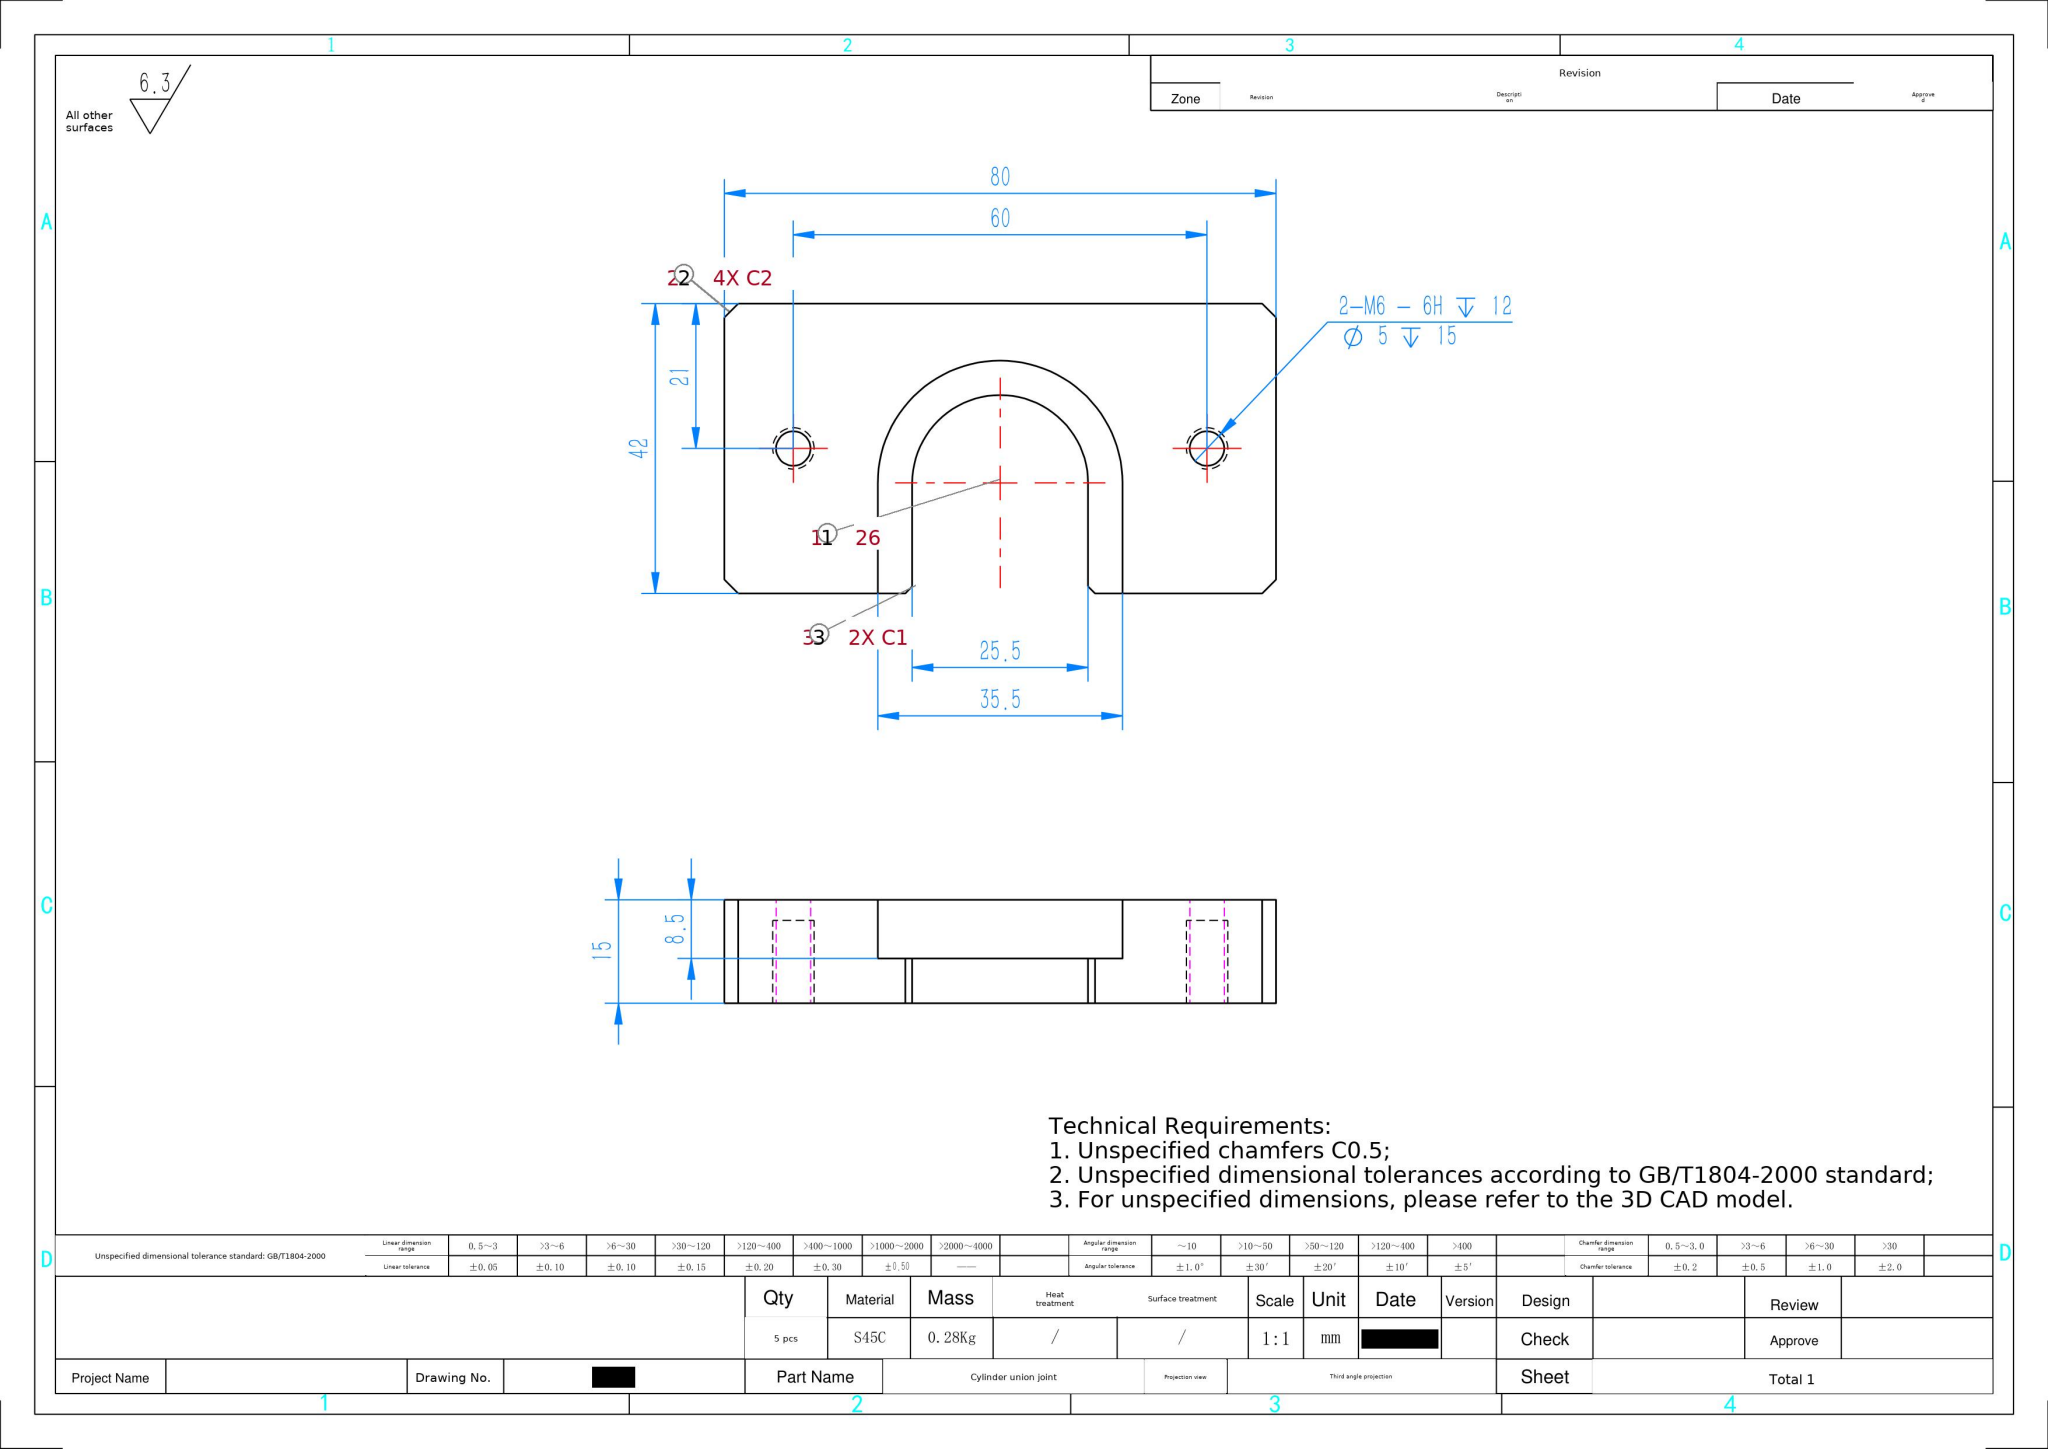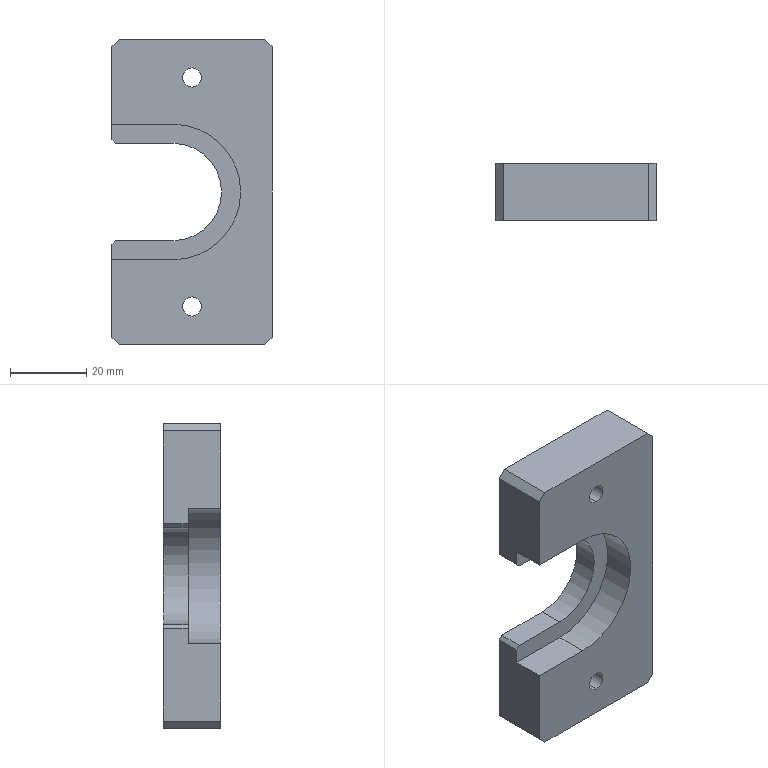Part | SolidWorks | mm | material S45C | 1 solid | 24 faces | box 42 x 15 x 80 mm | volume 36338 mm3 | plane 18 | cylinder 6 | commonest cylinder face diameters 5 x4 25.5 x1 35.5 x1
build123d program:
from build123d import *

# Parameters (mm, degrees)
SKETCH1_W             = 42
SKETCH1_H             = 80
BOSS_EXTRUDE1_DEPTH   = 15
CUT_EXTRUDE1_DEPTH    = 48.603
CUT_EXTRUDE2_DEPTH    = 8.5
M6_TAPPED_HOLE1_D     = 5
M6_TAPPED_HOLE1_DEPTH = 15
M6_TAPPED_HOLE1_TIP   = 1.502
CHAMFER1_SIZE         = 2
CHAMFER2_SIZE         = 1


with BuildPart() as part:
    # Sketch1 → Boss-Extrude1 (new body)
    with BuildSketch(Plane(origin=(0, 0, 0), x_dir=(1, 0, 0), z_dir=(0, 1, 0))):
        Rectangle(SKETCH1_W, SKETCH1_H)
    extrude(amount=BOSS_EXTRUDE1_DEPTH)

    # Sketch2 → Cut-Extrude1 (cut, through all)
    with BuildSketch(Plane(origin=(0, 15, 0), x_dir=(1, 0, 0), z_dir=(0, 1, 0))):
        with BuildLine():
            Line((-37, 12.75), (-5, 12.75))
            ThreePointArc((-5, 12.75), (7.75, 0), (-5, -12.75))
            Line((-5, -12.75), (-37, -12.75))
            ThreePointArc((-37, -12.75), (-49.75, 0), (-37, 12.75))
        make_face()
    extrude(amount=-CUT_EXTRUDE1_DEPTH, mode=Mode.SUBTRACT)

    # Sketch3 → Cut-Extrude2 (cut)
    with BuildSketch(Plane.XZ):
        with BuildLine():
            Line((-21, -17.75), (-21, 17.75))
            Line((-21, 17.75), (-5, 17.75))
            ThreePointArc((-5, 17.75), (12.75, 0), (-5, -17.75))
            Line((-5, -17.75), (-21, -17.75))
        make_face()
    extrude(amount=-CUT_EXTRUDE2_DEPTH, mode=Mode.SUBTRACT)

    # M6 Tapped Hole1
    with Locations(Plane(origin=(0, 15, 0), x_dir=(1, 0, 0), z_dir=(0, 1, 0))):
        with Locations((0, -30), (0, 30)):
            Hole(M6_TAPPED_HOLE1_D / 2, depth=M6_TAPPED_HOLE1_DEPTH)
            with Locations((0, 0, -(M6_TAPPED_HOLE1_DEPTH + M6_TAPPED_HOLE1_TIP / 2))):  # 118° drill point
                Cone(0, M6_TAPPED_HOLE1_D / 2, M6_TAPPED_HOLE1_TIP, mode=Mode.SUBTRACT)

    # Chamfer1
    chamfer1_edges = [part.edges().sort_by_distance(p)[0] for p in [
        (21, 7.5, 40),
        (-21, 7.5, 40),
        (-21, 7.5, -40),
        (21, 7.5, -40),
    ]]
    chamfer(chamfer1_edges, length=CHAMFER1_SIZE)

    # Chamfer2
    chamfer2_edges = [part.edges().sort_by_distance(p)[0] for p in [
        (-21, 11.75, 12.75),
        (-21, 11.75, -12.75),
    ]]
    chamfer(chamfer2_edges, length=CHAMFER2_SIZE)


solid = part.part
STEP:
#1=CARTESIAN_POINT('',(0.,0.,-32.5));
#2=VERTEX_POINT('',#1);
#3=CARTESIAN_POINT('',(0.,0.,-27.5));
#4=VERTEX_POINT('',#3);
#5=CARTESIAN_POINT('',(0.,0.,-30.));
#6=DIRECTION('',(0.,1.,0.));
#7=DIRECTION('',(0.,0.,1.));
#8=AXIS2_PLACEMENT_3D('',#5,#6,#7);
#9=CIRCLE('',#8,2.5);
#10=EDGE_CURVE('',#2,#4,#9,.T.);
#11=ORIENTED_EDGE('',*,*,#10,.F.);
#12=CARTESIAN_POINT('',(0.,15.,-32.5));
#13=VERTEX_POINT('',#12);
#14=CARTESIAN_POINT('',(0.,15.,-32.5));
#15=DIRECTION('',(0.,1.,0.));
#16=VECTOR('',#15,1000.);
#17=LINE('',#14,#16);
#18=EDGE_CURVE('',#2,#13,#17,.T.);
#19=ORIENTED_EDGE('',*,*,#18,.T.);
#20=CARTESIAN_POINT('',(0.,15.,-27.5));
#21=VERTEX_POINT('',#20);
#22=CARTESIAN_POINT('',(0.,15.,-30.));
#23=DIRECTION('',(0.,1.,0.));
#24=DIRECTION('',(0.,0.,1.));
#25=AXIS2_PLACEMENT_3D('',#22,#23,#24);
#26=CIRCLE('',#25,2.5);
#27=EDGE_CURVE('',#13,#21,#26,.T.);
#28=ORIENTED_EDGE('',*,*,#27,.T.);
#29=CARTESIAN_POINT('',(0.,15.,-27.5));
#30=DIRECTION('',(0.,1.,0.));
#31=VECTOR('',#30,1000.);
#32=LINE('',#29,#31);
#33=EDGE_CURVE('',#4,#21,#32,.T.);
#34=ORIENTED_EDGE('',*,*,#33,.F.);
#35=EDGE_LOOP('',(#11,#19,#28,#34));
#36=FACE_OUTER_BOUND('',#35,.T.);
#37=CARTESIAN_POINT('',(0.,15.,-30.));
#38=DIRECTION('',(0.,1.,0.));
#39=DIRECTION('',(0.,0.,1.));
#40=AXIS2_PLACEMENT_3D('',#37,#38,#39);
#41=CYLINDRICAL_SURFACE('',#40,2.5);
#42=ADVANCED_FACE('',(#36),#41,.F.);
#43=CARTESIAN_POINT('',(0.,0.,27.5));
#44=VERTEX_POINT('',#43);
#45=CARTESIAN_POINT('',(0.,0.,32.5));
#46=VERTEX_POINT('',#45);
#47=CARTESIAN_POINT('',(0.,0.,30.));
#48=DIRECTION('',(0.,1.,0.));
#49=DIRECTION('',(0.,0.,1.));
#50=AXIS2_PLACEMENT_3D('',#47,#48,#49);
#51=CIRCLE('',#50,2.5);
#52=EDGE_CURVE('',#44,#46,#51,.T.);
#53=ORIENTED_EDGE('',*,*,#52,.F.);
#54=CARTESIAN_POINT('',(0.,15.,27.5));
#55=VERTEX_POINT('',#54);
#56=CARTESIAN_POINT('',(0.,15.,27.5));
#57=DIRECTION('',(0.,1.,0.));
#58=VECTOR('',#57,1000.);
#59=LINE('',#56,#58);
#60=EDGE_CURVE('',#44,#55,#59,.T.);
#61=ORIENTED_EDGE('',*,*,#60,.T.);
#62=CARTESIAN_POINT('',(0.,15.,32.5));
#63=VERTEX_POINT('',#62);
#64=CARTESIAN_POINT('',(0.,15.,30.));
#65=DIRECTION('',(0.,1.,0.));
#66=DIRECTION('',(0.,0.,1.));
#67=AXIS2_PLACEMENT_3D('',#64,#65,#66);
#68=CIRCLE('',#67,2.5);
#69=EDGE_CURVE('',#55,#63,#68,.T.);
#70=ORIENTED_EDGE('',*,*,#69,.T.);
#71=CARTESIAN_POINT('',(0.,15.,32.5));
#72=DIRECTION('',(0.,1.,0.));
#73=VECTOR('',#72,1000.);
#74=LINE('',#71,#73);
#75=EDGE_CURVE('',#46,#63,#74,.T.);
#76=ORIENTED_EDGE('',*,*,#75,.F.);
#77=EDGE_LOOP('',(#53,#61,#70,#76));
#78=FACE_OUTER_BOUND('',#77,.T.);
#79=CARTESIAN_POINT('',(0.,15.,30.));
#80=DIRECTION('',(0.,1.,0.));
#81=DIRECTION('',(0.,0.,1.));
#82=AXIS2_PLACEMENT_3D('',#79,#80,#81);
#83=CYLINDRICAL_SURFACE('',#82,2.5);
#84=ADVANCED_FACE('',(#78),#83,.F.);
#85=CARTESIAN_POINT('',(-5.,15.,-12.75));
#86=VERTEX_POINT('',#85);
#87=CARTESIAN_POINT('',(-20.,15.,-12.75));
#88=VERTEX_POINT('',#87);
#89=CARTESIAN_POINT('',(-37.,15.,-12.75));
#90=DIRECTION('',(-1.,0.,0.));
#91=VECTOR('',#90,1000.);
#92=LINE('',#89,#91);
#93=EDGE_CURVE('',#86,#88,#92,.T.);
#94=ORIENTED_EDGE('',*,*,#93,.T.);
#95=CARTESIAN_POINT('',(-20.,8.5,-12.75));
#96=VERTEX_POINT('',#95);
#97=CARTESIAN_POINT('',(-20.,0.,-12.75));
#98=DIRECTION('',(0.,-1.,0.));
#99=VECTOR('',#98,1000.);
#100=LINE('',#97,#99);
#101=EDGE_CURVE('',#88,#96,#100,.T.);
#102=ORIENTED_EDGE('',*,*,#101,.T.);
#103=CARTESIAN_POINT('',(-5.,8.5,-12.75));
#104=VERTEX_POINT('',#103);
#105=CARTESIAN_POINT('',(-37.,8.5,-12.75));
#106=DIRECTION('',(-1.,0.,0.));
#107=VECTOR('',#106,1000.);
#108=LINE('',#105,#107);
#109=EDGE_CURVE('',#104,#96,#108,.T.);
#110=ORIENTED_EDGE('',*,*,#109,.F.);
#111=CARTESIAN_POINT('',(-5.,0.,-12.75));
#112=DIRECTION('',(0.,1.,0.));
#113=VECTOR('',#112,1000.);
#114=LINE('',#111,#113);
#115=EDGE_CURVE('',#104,#86,#114,.T.);
#116=ORIENTED_EDGE('',*,*,#115,.T.);
#117=EDGE_LOOP('',(#94,#102,#110,#116));
#118=FACE_OUTER_BOUND('',#117,.T.);
#119=CARTESIAN_POINT('',(-37.,0.,-12.75));
#120=DIRECTION('',(-0.,0.,-1.));
#121=DIRECTION('',(-1.,0.,0.));
#122=AXIS2_PLACEMENT_3D('',#119,#120,#121);
#123=PLANE('',#122);
#124=ADVANCED_FACE('',(#118),#123,.F.);
#125=CARTESIAN_POINT('',(-20.,8.5,12.75));
#126=VERTEX_POINT('',#125);
#127=CARTESIAN_POINT('',(-5.,8.5,12.75));
#128=VERTEX_POINT('',#127);
#129=CARTESIAN_POINT('',(-37.,8.5,12.75));
#130=DIRECTION('',(1.,0.,-0.));
#131=VECTOR('',#130,1000.);
#132=LINE('',#129,#131);
#133=EDGE_CURVE('',#126,#128,#132,.T.);
#134=ORIENTED_EDGE('',*,*,#133,.F.);
#135=CARTESIAN_POINT('',(-20.,15.,12.75));
#136=VERTEX_POINT('',#135);
#137=CARTESIAN_POINT('',(-20.,0.,12.75));
#138=DIRECTION('',(0.,1.,0.));
#139=VECTOR('',#138,1000.);
#140=LINE('',#137,#139);
#141=EDGE_CURVE('',#126,#136,#140,.T.);
#142=ORIENTED_EDGE('',*,*,#141,.T.);
#143=CARTESIAN_POINT('',(-5.,15.,12.75));
#144=VERTEX_POINT('',#143);
#145=CARTESIAN_POINT('',(-37.,15.,12.75));
#146=DIRECTION('',(1.,0.,-0.));
#147=VECTOR('',#146,1000.);
#148=LINE('',#145,#147);
#149=EDGE_CURVE('',#136,#144,#148,.T.);
#150=ORIENTED_EDGE('',*,*,#149,.T.);
#151=CARTESIAN_POINT('',(-5.,0.,12.75));
#152=DIRECTION('',(0.,1.,0.));
#153=VECTOR('',#152,1000.);
#154=LINE('',#151,#153);
#155=EDGE_CURVE('',#128,#144,#154,.T.);
#156=ORIENTED_EDGE('',*,*,#155,.F.);
#157=EDGE_LOOP('',(#134,#142,#150,#156));
#158=FACE_OUTER_BOUND('',#157,.T.);
#159=CARTESIAN_POINT('',(-37.,0.,12.75));
#160=DIRECTION('',(0.,0.,1.));
#161=DIRECTION('',(1.,0.,-0.));
#162=AXIS2_PLACEMENT_3D('',#159,#160,#161);
#163=PLANE('',#162);
#164=ADVANCED_FACE('',(#158),#163,.F.);
#165=CARTESIAN_POINT('',(-5.,8.5,-0.));
#166=DIRECTION('',(0.,1.,0.));
#167=DIRECTION('',(0.,0.,-1.));
#168=AXIS2_PLACEMENT_3D('',#165,#166,#167);
#169=CIRCLE('',#168,12.75);
#170=EDGE_CURVE('',#128,#104,#169,.T.);
#171=ORIENTED_EDGE('',*,*,#170,.F.);
#172=ORIENTED_EDGE('',*,*,#155,.T.);
#173=CARTESIAN_POINT('',(-5.,15.,-0.));
#174=DIRECTION('',(0.,1.,0.));
#175=DIRECTION('',(0.,0.,1.));
#176=AXIS2_PLACEMENT_3D('',#173,#174,#175);
#177=CIRCLE('',#176,12.75);
#178=EDGE_CURVE('',#144,#86,#177,.T.);
#179=ORIENTED_EDGE('',*,*,#178,.T.);
#180=ORIENTED_EDGE('',*,*,#115,.F.);
#181=EDGE_LOOP('',(#171,#172,#179,#180));
#182=FACE_OUTER_BOUND('',#181,.T.);
#183=CARTESIAN_POINT('',(-5.,0.,-0.));
#184=DIRECTION('',(0.,1.,0.));
#185=DIRECTION('',(0.,0.,1.));
#186=AXIS2_PLACEMENT_3D('',#183,#184,#185);
#187=CYLINDRICAL_SURFACE('',#186,12.75);
#188=ADVANCED_FACE('',(#182),#187,.F.);
#189=CARTESIAN_POINT('',(-21.,8.5,-13.75));
#190=VERTEX_POINT('',#189);
#191=CARTESIAN_POINT('',(-21.,8.5,-17.75));
#192=VERTEX_POINT('',#191);
#193=CARTESIAN_POINT('',(-21.,8.5,-17.75));
#194=DIRECTION('',(0.,0.,-1.));
#195=VECTOR('',#194,1000.);
#196=LINE('',#193,#195);
#197=EDGE_CURVE('',#190,#192,#196,.T.);
#198=ORIENTED_EDGE('',*,*,#197,.F.);
#199=CARTESIAN_POINT('',(-21.,15.,-13.75));
#200=VERTEX_POINT('',#199);
#201=CARTESIAN_POINT('',(-21.,15.,-13.75));
#202=DIRECTION('',(0.,1.,0.));
#203=VECTOR('',#202,1000.);
#204=LINE('',#201,#203);
#205=EDGE_CURVE('',#190,#200,#204,.T.);
#206=ORIENTED_EDGE('',*,*,#205,.T.);
#207=CARTESIAN_POINT('',(-21.,15.,-38.));
#208=VERTEX_POINT('',#207);
#209=CARTESIAN_POINT('',(-21.,15.,-40.));
#210=DIRECTION('',(0.,0.,1.));
#211=VECTOR('',#210,1000.);
#212=LINE('',#209,#211);
#213=EDGE_CURVE('',#208,#200,#212,.T.);
#214=ORIENTED_EDGE('',*,*,#213,.F.);
#215=CARTESIAN_POINT('',(-21.,0.,-38.));
#216=VERTEX_POINT('',#215);
#217=CARTESIAN_POINT('',(-21.,15.,-38.));
#218=DIRECTION('',(0.,-1.,0.));
#219=VECTOR('',#218,1000.);
#220=LINE('',#217,#219);
#221=EDGE_CURVE('',#208,#216,#220,.T.);
#222=ORIENTED_EDGE('',*,*,#221,.T.);
#223=CARTESIAN_POINT('',(-21.,0.,-17.75));
#224=VERTEX_POINT('',#223);
#225=CARTESIAN_POINT('',(-21.,0.,-40.));
#226=DIRECTION('',(0.,0.,1.));
#227=VECTOR('',#226,1000.);
#228=LINE('',#225,#227);
#229=EDGE_CURVE('',#216,#224,#228,.T.);
#230=ORIENTED_EDGE('',*,*,#229,.T.);
#231=CARTESIAN_POINT('',(-21.,8.5,-17.75));
#232=DIRECTION('',(0.,-1.,0.));
#233=VECTOR('',#232,1000.);
#234=LINE('',#231,#233);
#235=EDGE_CURVE('',#192,#224,#234,.T.);
#236=ORIENTED_EDGE('',*,*,#235,.F.);
#237=EDGE_LOOP('',(#198,#206,#214,#222,#230,#236));
#238=FACE_OUTER_BOUND('',#237,.T.);
#239=CARTESIAN_POINT('',(-21.,15.,-40.));
#240=DIRECTION('',(1.,0.,-0.));
#241=DIRECTION('',(-0.,0.,-1.));
#242=AXIS2_PLACEMENT_3D('',#239,#240,#241);
#243=PLANE('',#242);
#244=ADVANCED_FACE('',(#238),#243,.F.);
#245=CARTESIAN_POINT('',(21.,0.,38.));
#246=VERTEX_POINT('',#245);
#247=CARTESIAN_POINT('',(21.,0.,-38.));
#248=VERTEX_POINT('',#247);
#249=CARTESIAN_POINT('',(21.,0.,-40.));
#250=DIRECTION('',(-0.,0.,-1.));
#251=VECTOR('',#250,1000.);
#252=LINE('',#249,#251);
#253=EDGE_CURVE('',#246,#248,#252,.T.);
#254=ORIENTED_EDGE('',*,*,#253,.T.);
#255=CARTESIAN_POINT('',(21.,15.,-38.));
#256=VERTEX_POINT('',#255);
#257=CARTESIAN_POINT('',(21.,15.,-38.));
#258=DIRECTION('',(0.,1.,0.));
#259=VECTOR('',#258,1000.);
#260=LINE('',#257,#259);
#261=EDGE_CURVE('',#248,#256,#260,.T.);
#262=ORIENTED_EDGE('',*,*,#261,.T.);
#263=CARTESIAN_POINT('',(21.,15.,38.));
#264=VERTEX_POINT('',#263);
#265=CARTESIAN_POINT('',(21.,15.,-40.));
#266=DIRECTION('',(-0.,0.,-1.));
#267=VECTOR('',#266,1000.);
#268=LINE('',#265,#267);
#269=EDGE_CURVE('',#264,#256,#268,.T.);
#270=ORIENTED_EDGE('',*,*,#269,.F.);
#271=CARTESIAN_POINT('',(21.,15.,38.));
#272=DIRECTION('',(0.,-1.,0.));
#273=VECTOR('',#272,1000.);
#274=LINE('',#271,#273);
#275=EDGE_CURVE('',#264,#246,#274,.T.);
#276=ORIENTED_EDGE('',*,*,#275,.T.);
#277=EDGE_LOOP('',(#254,#262,#270,#276));
#278=FACE_OUTER_BOUND('',#277,.T.);
#279=CARTESIAN_POINT('',(21.,15.,-40.));
#280=DIRECTION('',(-1.,0.,0.));
#281=DIRECTION('',(0.,0.,1.));
#282=AXIS2_PLACEMENT_3D('',#279,#280,#281);
#283=PLANE('',#282);
#284=ADVANCED_FACE('',(#278),#283,.F.);
#285=CARTESIAN_POINT('',(19.,15.,-40.));
#286=VERTEX_POINT('',#285);
#287=CARTESIAN_POINT('',(-19.,15.,-40.));
#288=VERTEX_POINT('',#287);
#289=CARTESIAN_POINT('',(-21.,15.,-40.));
#290=DIRECTION('',(-1.,0.,0.));
#291=VECTOR('',#290,1000.);
#292=LINE('',#289,#291);
#293=EDGE_CURVE('',#286,#288,#292,.T.);
#294=ORIENTED_EDGE('',*,*,#293,.F.);
#295=CARTESIAN_POINT('',(19.,0.,-40.));
#296=VERTEX_POINT('',#295);
#297=CARTESIAN_POINT('',(19.,15.,-40.));
#298=DIRECTION('',(0.,-1.,0.));
#299=VECTOR('',#298,1000.);
#300=LINE('',#297,#299);
#301=EDGE_CURVE('',#286,#296,#300,.T.);
#302=ORIENTED_EDGE('',*,*,#301,.T.);
#303=CARTESIAN_POINT('',(-19.,0.,-40.));
#304=VERTEX_POINT('',#303);
#305=CARTESIAN_POINT('',(-21.,0.,-40.));
#306=DIRECTION('',(-1.,0.,0.));
#307=VECTOR('',#306,1000.);
#308=LINE('',#305,#307);
#309=EDGE_CURVE('',#296,#304,#308,.T.);
#310=ORIENTED_EDGE('',*,*,#309,.T.);
#311=CARTESIAN_POINT('',(-19.,15.,-40.));
#312=DIRECTION('',(0.,1.,0.));
#313=VECTOR('',#312,1000.);
#314=LINE('',#311,#313);
#315=EDGE_CURVE('',#304,#288,#314,.T.);
#316=ORIENTED_EDGE('',*,*,#315,.T.);
#317=EDGE_LOOP('',(#294,#302,#310,#316));
#318=FACE_OUTER_BOUND('',#317,.T.);
#319=CARTESIAN_POINT('',(-21.,15.,-40.));
#320=DIRECTION('',(0.,0.,1.));
#321=DIRECTION('',(1.,0.,0.));
#322=AXIS2_PLACEMENT_3D('',#319,#320,#321);
#323=PLANE('',#322);
#324=ADVANCED_FACE('',(#318),#323,.F.);
#325=CARTESIAN_POINT('',(-21.,15.,13.75));
#326=VERTEX_POINT('',#325);
#327=CARTESIAN_POINT('',(-21.,15.,38.));
#328=VERTEX_POINT('',#327);
#329=CARTESIAN_POINT('',(-21.,15.,-40.));
#330=DIRECTION('',(0.,0.,1.));
#331=VECTOR('',#330,1000.);
#332=LINE('',#329,#331);
#333=EDGE_CURVE('',#326,#328,#332,.T.);
#334=ORIENTED_EDGE('',*,*,#333,.F.);
#335=CARTESIAN_POINT('',(-21.,8.5,13.75));
#336=VERTEX_POINT('',#335);
#337=CARTESIAN_POINT('',(-21.,15.,13.75));
#338=DIRECTION('',(0.,-1.,0.));
#339=VECTOR('',#338,1000.);
#340=LINE('',#337,#339);
#341=EDGE_CURVE('',#326,#336,#340,.T.);
#342=ORIENTED_EDGE('',*,*,#341,.T.);
#343=CARTESIAN_POINT('',(-21.,8.5,17.75));
#344=VERTEX_POINT('',#343);
#345=CARTESIAN_POINT('',(-21.,8.5,-17.75));
#346=DIRECTION('',(0.,0.,-1.));
#347=VECTOR('',#346,1000.);
#348=LINE('',#345,#347);
#349=EDGE_CURVE('',#344,#336,#348,.T.);
#350=ORIENTED_EDGE('',*,*,#349,.F.);
#351=CARTESIAN_POINT('',(-21.,0.,17.75));
#352=VERTEX_POINT('',#351);
#353=CARTESIAN_POINT('',(-21.,8.5,17.75));
#354=DIRECTION('',(0.,-1.,0.));
#355=VECTOR('',#354,1000.);
#356=LINE('',#353,#355);
#357=EDGE_CURVE('',#344,#352,#356,.T.);
#358=ORIENTED_EDGE('',*,*,#357,.T.);
#359=CARTESIAN_POINT('',(-21.,0.,38.));
#360=VERTEX_POINT('',#359);
#361=CARTESIAN_POINT('',(-21.,0.,-40.));
#362=DIRECTION('',(0.,0.,1.));
#363=VECTOR('',#362,1000.);
#364=LINE('',#361,#363);
#365=EDGE_CURVE('',#352,#360,#364,.T.);
#366=ORIENTED_EDGE('',*,*,#365,.T.);
#367=CARTESIAN_POINT('',(-21.,15.,38.));
#368=DIRECTION('',(0.,1.,0.));
#369=VECTOR('',#368,1000.);
#370=LINE('',#367,#369);
#371=EDGE_CURVE('',#360,#328,#370,.T.);
#372=ORIENTED_EDGE('',*,*,#371,.T.);
#373=EDGE_LOOP('',(#334,#342,#350,#358,#366,#372));
#374=FACE_OUTER_BOUND('',#373,.T.);
#375=CARTESIAN_POINT('',(-21.,15.,-40.));
#376=DIRECTION('',(1.,0.,-0.));
#377=DIRECTION('',(-0.,0.,-1.));
#378=AXIS2_PLACEMENT_3D('',#375,#376,#377);
#379=PLANE('',#378);
#380=ADVANCED_FACE('',(#374),#379,.F.);
#381=CARTESIAN_POINT('',(-19.,15.,40.));
#382=VERTEX_POINT('',#381);
#383=CARTESIAN_POINT('',(19.,15.,40.));
#384=VERTEX_POINT('',#383);
#385=CARTESIAN_POINT('',(-21.,15.,40.));
#386=DIRECTION('',(1.,0.,0.));
#387=VECTOR('',#386,1000.);
#388=LINE('',#385,#387);
#389=EDGE_CURVE('',#382,#384,#388,.T.);
#390=ORIENTED_EDGE('',*,*,#389,.F.);
#391=CARTESIAN_POINT('',(-19.,0.,40.));
#392=VERTEX_POINT('',#391);
#393=CARTESIAN_POINT('',(-19.,15.,40.));
#394=DIRECTION('',(0.,-1.,0.));
#395=VECTOR('',#394,1000.);
#396=LINE('',#393,#395);
#397=EDGE_CURVE('',#382,#392,#396,.T.);
#398=ORIENTED_EDGE('',*,*,#397,.T.);
#399=CARTESIAN_POINT('',(19.,0.,40.));
#400=VERTEX_POINT('',#399);
#401=CARTESIAN_POINT('',(-21.,0.,40.));
#402=DIRECTION('',(1.,0.,0.));
#403=VECTOR('',#402,1000.);
#404=LINE('',#401,#403);
#405=EDGE_CURVE('',#392,#400,#404,.T.);
#406=ORIENTED_EDGE('',*,*,#405,.T.);
#407=CARTESIAN_POINT('',(19.,15.,40.));
#408=DIRECTION('',(0.,1.,0.));
#409=VECTOR('',#408,1000.);
#410=LINE('',#407,#409);
#411=EDGE_CURVE('',#400,#384,#410,.T.);
#412=ORIENTED_EDGE('',*,*,#411,.T.);
#413=EDGE_LOOP('',(#390,#398,#406,#412));
#414=FACE_OUTER_BOUND('',#413,.T.);
#415=CARTESIAN_POINT('',(-21.,15.,40.));
#416=DIRECTION('',(0.,0.,-1.));
#417=DIRECTION('',(-1.,0.,0.));
#418=AXIS2_PLACEMENT_3D('',#415,#416,#417);
#419=PLANE('',#418);
#420=ADVANCED_FACE('',(#414),#419,.F.);
#421=CARTESIAN_POINT('',(0.,15.,-30.));
#422=DIRECTION('',(0.,1.,0.));
#423=DIRECTION('',(0.,0.,1.));
#424=AXIS2_PLACEMENT_3D('',#421,#422,#423);
#425=CIRCLE('',#424,2.5);
#426=EDGE_CURVE('',#21,#13,#425,.T.);
#427=ORIENTED_EDGE('',*,*,#426,.F.);
#428=ORIENTED_EDGE('',*,*,#27,.F.);
#429=EDGE_LOOP('',(#427,#428));
#430=FACE_BOUND('',#429,.T.);
#431=CARTESIAN_POINT('',(0.,15.,30.));
#432=DIRECTION('',(0.,1.,0.));
#433=DIRECTION('',(0.,0.,1.));
#434=AXIS2_PLACEMENT_3D('',#431,#432,#433);
#435=CIRCLE('',#434,2.5);
#436=EDGE_CURVE('',#63,#55,#435,.T.);
#437=ORIENTED_EDGE('',*,*,#436,.F.);
#438=ORIENTED_EDGE('',*,*,#69,.F.);
#439=EDGE_LOOP('',(#437,#438));
#440=FACE_BOUND('',#439,.T.);
#441=ORIENTED_EDGE('',*,*,#213,.T.);
#442=CARTESIAN_POINT('',(-3.625,15.,3.625));
#443=DIRECTION('',(0.7071,0.,0.7071));
#444=VECTOR('',#443,1000.);
#445=LINE('',#442,#444);
#446=EDGE_CURVE('',#200,#88,#445,.T.);
#447=ORIENTED_EDGE('',*,*,#446,.T.);
#448=ORIENTED_EDGE('',*,*,#93,.F.);
#449=ORIENTED_EDGE('',*,*,#178,.F.);
#450=ORIENTED_EDGE('',*,*,#149,.F.);
#451=CARTESIAN_POINT('',(-3.625,15.,-3.625));
#452=DIRECTION('',(-0.7071,0.,0.7071));
#453=VECTOR('',#452,1000.);
#454=LINE('',#451,#453);
#455=EDGE_CURVE('',#136,#326,#454,.T.);
#456=ORIENTED_EDGE('',*,*,#455,.T.);
#457=ORIENTED_EDGE('',*,*,#333,.T.);
#458=CARTESIAN_POINT('',(-29.5,15.,29.5));
#459=DIRECTION('',(0.7071,0.,0.7071));
#460=VECTOR('',#459,1000.);
#461=LINE('',#458,#460);
#462=EDGE_CURVE('',#328,#382,#461,.T.);
#463=ORIENTED_EDGE('',*,*,#462,.T.);
#464=ORIENTED_EDGE('',*,*,#389,.T.);
#465=CARTESIAN_POINT('',(29.5,15.,29.5));
#466=DIRECTION('',(0.7071,0.,-0.7071));
#467=VECTOR('',#466,1000.);
#468=LINE('',#465,#467);
#469=EDGE_CURVE('',#384,#264,#468,.T.);
#470=ORIENTED_EDGE('',*,*,#469,.T.);
#471=ORIENTED_EDGE('',*,*,#269,.T.);
#472=CARTESIAN_POINT('',(29.5,15.,-29.5));
#473=DIRECTION('',(-0.7071,0.,-0.7071));
#474=VECTOR('',#473,1000.);
#475=LINE('',#472,#474);
#476=EDGE_CURVE('',#256,#286,#475,.T.);
#477=ORIENTED_EDGE('',*,*,#476,.T.);
#478=ORIENTED_EDGE('',*,*,#293,.T.);
#479=CARTESIAN_POINT('',(-29.5,15.,-29.5));
#480=DIRECTION('',(-0.7071,0.,0.7071));
#481=VECTOR('',#480,1000.);
#482=LINE('',#479,#481);
#483=EDGE_CURVE('',#288,#208,#482,.T.);
#484=ORIENTED_EDGE('',*,*,#483,.T.);
#485=EDGE_LOOP('',(#441,#447,#448,#449,#450,#456,#457,#463,#464,#470,#471,#477,#478,#484));
#486=FACE_OUTER_BOUND('',#485,.T.);
#487=CARTESIAN_POINT('',(0.,15.,0.));
#488=DIRECTION('',(0.,1.,0.));
#489=DIRECTION('',(0.,0.,1.));
#490=AXIS2_PLACEMENT_3D('',#487,#488,#489);
#491=PLANE('',#490);
#492=ADVANCED_FACE('',(#430,#440,#486),#491,.T.);
#493=CARTESIAN_POINT('',(0.,0.,-30.));
#494=DIRECTION('',(0.,1.,0.));
#495=DIRECTION('',(0.,0.,1.));
#496=AXIS2_PLACEMENT_3D('',#493,#494,#495);
#497=CIRCLE('',#496,2.5);
#498=EDGE_CURVE('',#4,#2,#497,.T.);
#499=ORIENTED_EDGE('',*,*,#498,.T.);
#500=ORIENTED_EDGE('',*,*,#10,.T.);
#501=EDGE_LOOP('',(#499,#500));
#502=FACE_BOUND('',#501,.T.);
#503=CARTESIAN_POINT('',(0.,0.,30.));
#504=DIRECTION('',(0.,1.,0.));
#505=DIRECTION('',(0.,0.,1.));
#506=AXIS2_PLACEMENT_3D('',#503,#504,#505);
#507=CIRCLE('',#506,2.5);
#508=EDGE_CURVE('',#46,#44,#507,.T.);
#509=ORIENTED_EDGE('',*,*,#508,.T.);
#510=ORIENTED_EDGE('',*,*,#52,.T.);
#511=EDGE_LOOP('',(#509,#510));
#512=FACE_BOUND('',#511,.T.);
#513=ORIENTED_EDGE('',*,*,#309,.F.);
#514=CARTESIAN_POINT('',(19.,0.,-40.));
#515=DIRECTION('',(0.7071,0.,0.7071));
#516=VECTOR('',#515,1000.);
#517=LINE('',#514,#516);
#518=EDGE_CURVE('',#296,#248,#517,.T.);
#519=ORIENTED_EDGE('',*,*,#518,.T.);
#520=ORIENTED_EDGE('',*,*,#253,.F.);
#521=CARTESIAN_POINT('',(21.,0.,38.));
#522=DIRECTION('',(-0.7071,0.,0.7071));
#523=VECTOR('',#522,1000.);
#524=LINE('',#521,#523);
#525=EDGE_CURVE('',#246,#400,#524,.T.);
#526=ORIENTED_EDGE('',*,*,#525,.T.);
#527=ORIENTED_EDGE('',*,*,#405,.F.);
#528=CARTESIAN_POINT('',(-19.,0.,40.));
#529=DIRECTION('',(-0.7071,0.,-0.7071));
#530=VECTOR('',#529,1000.);
#531=LINE('',#528,#530);
#532=EDGE_CURVE('',#392,#360,#531,.T.);
#533=ORIENTED_EDGE('',*,*,#532,.T.);
#534=ORIENTED_EDGE('',*,*,#365,.F.);
#535=CARTESIAN_POINT('',(-5.,0.,17.75));
#536=VERTEX_POINT('',#535);
#537=CARTESIAN_POINT('',(-21.,0.,17.75));
#538=DIRECTION('',(-1.,0.,0.));
#539=VECTOR('',#538,1000.);
#540=LINE('',#537,#539);
#541=EDGE_CURVE('',#536,#352,#540,.T.);
#542=ORIENTED_EDGE('',*,*,#541,.F.);
#543=CARTESIAN_POINT('',(-5.,0.,-17.75));
#544=VERTEX_POINT('',#543);
#545=CARTESIAN_POINT('',(-5.,0.,-0.));
#546=DIRECTION('',(0.,-1.,0.));
#547=DIRECTION('',(0.,0.,-1.));
#548=AXIS2_PLACEMENT_3D('',#545,#546,#547);
#549=CIRCLE('',#548,17.75);
#550=EDGE_CURVE('',#544,#536,#549,.T.);
#551=ORIENTED_EDGE('',*,*,#550,.F.);
#552=CARTESIAN_POINT('',(-5.,0.,-17.75));
#553=DIRECTION('',(1.,0.,0.));
#554=VECTOR('',#553,1000.);
#555=LINE('',#552,#554);
#556=EDGE_CURVE('',#224,#544,#555,.T.);
#557=ORIENTED_EDGE('',*,*,#556,.F.);
#558=ORIENTED_EDGE('',*,*,#229,.F.);
#559=CARTESIAN_POINT('',(-21.,0.,-38.));
#560=DIRECTION('',(0.7071,0.,-0.7071));
#561=VECTOR('',#560,1000.);
#562=LINE('',#559,#561);
#563=EDGE_CURVE('',#216,#304,#562,.T.);
#564=ORIENTED_EDGE('',*,*,#563,.T.);
#565=EDGE_LOOP('',(#513,#519,#520,#526,#527,#533,#534,#542,#551,#557,#558,#564));
#566=FACE_OUTER_BOUND('',#565,.T.);
#567=CARTESIAN_POINT('',(0.,0.,0.));
#568=DIRECTION('',(0.,1.,0.));
#569=DIRECTION('',(0.,0.,1.));
#570=AXIS2_PLACEMENT_3D('',#567,#568,#569);
#571=PLANE('',#570);
#572=ADVANCED_FACE('',(#502,#512,#566),#571,.F.);
#573=ORIENTED_EDGE('',*,*,#109,.T.);
#574=CARTESIAN_POINT('',(-6.125,8.5,1.125));
#575=DIRECTION('',(-0.7071,0.,-0.7071));
#576=VECTOR('',#575,1000.);
#577=LINE('',#574,#576);
#578=EDGE_CURVE('',#96,#190,#577,.T.);
#579=ORIENTED_EDGE('',*,*,#578,.T.);
#580=ORIENTED_EDGE('',*,*,#197,.T.);
#581=CARTESIAN_POINT('',(-5.,8.5,-17.75));
#582=VERTEX_POINT('',#581);
#583=CARTESIAN_POINT('',(-5.,8.5,-17.75));
#584=DIRECTION('',(1.,0.,0.));
#585=VECTOR('',#584,1000.);
#586=LINE('',#583,#585);
#587=EDGE_CURVE('',#192,#582,#586,.T.);
#588=ORIENTED_EDGE('',*,*,#587,.T.);
#589=CARTESIAN_POINT('',(-5.,8.5,17.75));
#590=VERTEX_POINT('',#589);
#591=CARTESIAN_POINT('',(-5.,8.5,-0.));
#592=DIRECTION('',(0.,-1.,0.));
#593=DIRECTION('',(0.,0.,-1.));
#594=AXIS2_PLACEMENT_3D('',#591,#592,#593);
#595=CIRCLE('',#594,17.75);
#596=EDGE_CURVE('',#582,#590,#595,.T.);
#597=ORIENTED_EDGE('',*,*,#596,.T.);
#598=CARTESIAN_POINT('',(-21.,8.5,17.75));
#599=DIRECTION('',(-1.,0.,0.));
#600=VECTOR('',#599,1000.);
#601=LINE('',#598,#600);
#602=EDGE_CURVE('',#590,#344,#601,.T.);
#603=ORIENTED_EDGE('',*,*,#602,.T.);
#604=ORIENTED_EDGE('',*,*,#349,.T.);
#605=CARTESIAN_POINT('',(-6.125,8.5,-1.125));
#606=DIRECTION('',(0.7071,0.,-0.7071));
#607=VECTOR('',#606,1000.);
#608=LINE('',#605,#607);
#609=EDGE_CURVE('',#336,#126,#608,.T.);
#610=ORIENTED_EDGE('',*,*,#609,.T.);
#611=ORIENTED_EDGE('',*,*,#133,.T.);
#612=ORIENTED_EDGE('',*,*,#170,.T.);
#613=EDGE_LOOP('',(#573,#579,#580,#588,#597,#603,#604,#610,#611,#612));
#614=FACE_OUTER_BOUND('',#613,.T.);
#615=CARTESIAN_POINT('',(-5.,8.5,-0.));
#616=DIRECTION('',(0.,-1.,0.));
#617=DIRECTION('',(0.,0.,-1.));
#618=AXIS2_PLACEMENT_3D('',#615,#616,#617);
#619=PLANE('',#618);
#620=ADVANCED_FACE('',(#614),#619,.T.);
#621=ORIENTED_EDGE('',*,*,#550,.T.);
#622=CARTESIAN_POINT('',(-5.,8.5,17.75));
#623=DIRECTION('',(0.,-1.,0.));
#624=VECTOR('',#623,1000.);
#625=LINE('',#622,#624);
#626=EDGE_CURVE('',#590,#536,#625,.T.);
#627=ORIENTED_EDGE('',*,*,#626,.F.);
#628=ORIENTED_EDGE('',*,*,#596,.F.);
#629=CARTESIAN_POINT('',(-5.,8.5,-17.75));
#630=DIRECTION('',(0.,-1.,0.));
#631=VECTOR('',#630,1000.);
#632=LINE('',#629,#631);
#633=EDGE_CURVE('',#582,#544,#632,.T.);
#634=ORIENTED_EDGE('',*,*,#633,.T.);
#635=EDGE_LOOP('',(#621,#627,#628,#634));
#636=FACE_OUTER_BOUND('',#635,.T.);
#637=CARTESIAN_POINT('',(-5.,8.5,-0.));
#638=DIRECTION('',(0.,-1.,0.));
#639=DIRECTION('',(0.,0.,-1.));
#640=AXIS2_PLACEMENT_3D('',#637,#638,#639);
#641=CYLINDRICAL_SURFACE('',#640,17.75);
#642=ADVANCED_FACE('',(#636),#641,.F.);
#643=ORIENTED_EDGE('',*,*,#556,.T.);
#644=ORIENTED_EDGE('',*,*,#633,.F.);
#645=ORIENTED_EDGE('',*,*,#587,.F.);
#646=ORIENTED_EDGE('',*,*,#235,.T.);
#647=EDGE_LOOP('',(#643,#644,#645,#646));
#648=FACE_OUTER_BOUND('',#647,.T.);
#649=CARTESIAN_POINT('',(-5.,8.5,-17.75));
#650=DIRECTION('',(0.,0.,-1.));
#651=DIRECTION('',(-1.,0.,-0.));
#652=AXIS2_PLACEMENT_3D('',#649,#650,#651);
#653=PLANE('',#652);
#654=ADVANCED_FACE('',(#648),#653,.F.);
#655=ORIENTED_EDGE('',*,*,#541,.T.);
#656=ORIENTED_EDGE('',*,*,#357,.F.);
#657=ORIENTED_EDGE('',*,*,#602,.F.);
#658=ORIENTED_EDGE('',*,*,#626,.T.);
#659=EDGE_LOOP('',(#655,#656,#657,#658));
#660=FACE_OUTER_BOUND('',#659,.T.);
#661=CARTESIAN_POINT('',(-21.,8.5,17.75));
#662=DIRECTION('',(0.,0.,1.));
#663=DIRECTION('',(1.,0.,-0.));
#664=AXIS2_PLACEMENT_3D('',#661,#662,#663);
#665=PLANE('',#664);
#666=ADVANCED_FACE('',(#660),#665,.F.);
#667=ORIENTED_EDGE('',*,*,#60,.F.);
#668=ORIENTED_EDGE('',*,*,#508,.F.);
#669=ORIENTED_EDGE('',*,*,#75,.T.);
#670=ORIENTED_EDGE('',*,*,#436,.T.);
#671=EDGE_LOOP('',(#667,#668,#669,#670));
#672=FACE_OUTER_BOUND('',#671,.T.);
#673=CARTESIAN_POINT('',(0.,15.,30.));
#674=DIRECTION('',(0.,1.,0.));
#675=DIRECTION('',(0.,0.,1.));
#676=AXIS2_PLACEMENT_3D('',#673,#674,#675);
#677=CYLINDRICAL_SURFACE('',#676,2.5);
#678=ADVANCED_FACE('',(#672),#677,.F.);
#679=ORIENTED_EDGE('',*,*,#18,.F.);
#680=ORIENTED_EDGE('',*,*,#498,.F.);
#681=ORIENTED_EDGE('',*,*,#33,.T.);
#682=ORIENTED_EDGE('',*,*,#426,.T.);
#683=EDGE_LOOP('',(#679,#680,#681,#682));
#684=FACE_OUTER_BOUND('',#683,.T.);
#685=CARTESIAN_POINT('',(0.,15.,-30.));
#686=DIRECTION('',(0.,1.,0.));
#687=DIRECTION('',(0.,0.,1.));
#688=AXIS2_PLACEMENT_3D('',#685,#686,#687);
#689=CYLINDRICAL_SURFACE('',#688,2.5);
#690=ADVANCED_FACE('',(#684),#689,.F.);
#691=ORIENTED_EDGE('',*,*,#476,.F.);
#692=ORIENTED_EDGE('',*,*,#261,.F.);
#693=ORIENTED_EDGE('',*,*,#518,.F.);
#694=ORIENTED_EDGE('',*,*,#301,.F.);
#695=EDGE_LOOP('',(#691,#692,#693,#694));
#696=FACE_OUTER_BOUND('',#695,.T.);
#697=CARTESIAN_POINT('',(19.,15.,-40.));
#698=DIRECTION('',(-0.7071,0.,0.7071));
#699=DIRECTION('',(0.,-1.,0.));
#700=AXIS2_PLACEMENT_3D('',#697,#698,#699);
#701=PLANE('',#700);
#702=ADVANCED_FACE('',(#696),#701,.F.);
#703=ORIENTED_EDGE('',*,*,#483,.F.);
#704=ORIENTED_EDGE('',*,*,#315,.F.);
#705=ORIENTED_EDGE('',*,*,#563,.F.);
#706=ORIENTED_EDGE('',*,*,#221,.F.);
#707=EDGE_LOOP('',(#703,#704,#705,#706));
#708=FACE_OUTER_BOUND('',#707,.T.);
#709=CARTESIAN_POINT('',(-21.,15.,-38.));
#710=DIRECTION('',(0.7071,0.,0.7071));
#711=DIRECTION('',(0.,-1.,0.));
#712=AXIS2_PLACEMENT_3D('',#709,#710,#711);
#713=PLANE('',#712);
#714=ADVANCED_FACE('',(#708),#713,.F.);
#715=ORIENTED_EDGE('',*,*,#462,.F.);
#716=ORIENTED_EDGE('',*,*,#371,.F.);
#717=ORIENTED_EDGE('',*,*,#532,.F.);
#718=ORIENTED_EDGE('',*,*,#397,.F.);
#719=EDGE_LOOP('',(#715,#716,#717,#718));
#720=FACE_OUTER_BOUND('',#719,.T.);
#721=CARTESIAN_POINT('',(-19.,15.,40.));
#722=DIRECTION('',(0.7071,0.,-0.7071));
#723=DIRECTION('',(0.,-1.,0.));
#724=AXIS2_PLACEMENT_3D('',#721,#722,#723);
#725=PLANE('',#724);
#726=ADVANCED_FACE('',(#720),#725,.F.);
#727=ORIENTED_EDGE('',*,*,#469,.F.);
#728=ORIENTED_EDGE('',*,*,#411,.F.);
#729=ORIENTED_EDGE('',*,*,#525,.F.);
#730=ORIENTED_EDGE('',*,*,#275,.F.);
#731=EDGE_LOOP('',(#727,#728,#729,#730));
#732=FACE_OUTER_BOUND('',#731,.T.);
#733=CARTESIAN_POINT('',(21.,15.,38.));
#734=DIRECTION('',(-0.7071,0.,-0.7071));
#735=DIRECTION('',(0.,-1.,0.));
#736=AXIS2_PLACEMENT_3D('',#733,#734,#735);
#737=PLANE('',#736);
#738=ADVANCED_FACE('',(#732),#737,.F.);
#739=ORIENTED_EDGE('',*,*,#578,.F.);
#740=ORIENTED_EDGE('',*,*,#101,.F.);
#741=ORIENTED_EDGE('',*,*,#446,.F.);
#742=ORIENTED_EDGE('',*,*,#205,.F.);
#743=EDGE_LOOP('',(#739,#740,#741,#742));
#744=FACE_OUTER_BOUND('',#743,.T.);
#745=CARTESIAN_POINT('',(-21.,15.,-13.75));
#746=DIRECTION('',(0.7071,0.,-0.7071));
#747=DIRECTION('',(0.,1.,0.));
#748=AXIS2_PLACEMENT_3D('',#745,#746,#747);
#749=PLANE('',#748);
#750=ADVANCED_FACE('',(#744),#749,.F.);
#751=ORIENTED_EDGE('',*,*,#455,.F.);
#752=ORIENTED_EDGE('',*,*,#141,.F.);
#753=ORIENTED_EDGE('',*,*,#609,.F.);
#754=ORIENTED_EDGE('',*,*,#341,.F.);
#755=EDGE_LOOP('',(#751,#752,#753,#754));
#756=FACE_OUTER_BOUND('',#755,.T.);
#757=CARTESIAN_POINT('',(-21.,15.,13.75));
#758=DIRECTION('',(0.7071,0.,0.7071));
#759=DIRECTION('',(0.,-1.,0.));
#760=AXIS2_PLACEMENT_3D('',#757,#758,#759);
#761=PLANE('',#760);
#762=ADVANCED_FACE('',(#756),#761,.F.);
#763=CLOSED_SHELL('',(#42,#84,#124,#164,#188,#244,#284,#324,#380,#420,#492,#572,#620,#642,#654,#666,#678,#690,#702,#714,#726,#738,#750,#762));
#764=MANIFOLD_SOLID_BREP('',#763);
#765=CARTESIAN_POINT('',(0.,0.,0.));
#766=DIRECTION('',(0.,0.,1.));
#767=DIRECTION('',(1.,0.,0.));
#768=AXIS2_PLACEMENT_3D('',#765,#766,#767);
#769=(LENGTH_UNIT()NAMED_UNIT(*)SI_UNIT(.MILLI.,.METRE.));
#770=UNCERTAINTY_MEASURE_WITH_UNIT(LENGTH_MEASURE(0.00001),#769,'','');
#771=(NAMED_UNIT(*)PLANE_ANGLE_UNIT()SI_UNIT($,.RADIAN.));
#772=(NAMED_UNIT(*)SI_UNIT($,.STERADIAN.)SOLID_ANGLE_UNIT());
#773=(GEOMETRIC_REPRESENTATION_CONTEXT(3)GLOBAL_UNCERTAINTY_ASSIGNED_CONTEXT((#770))GLOBAL_UNIT_ASSIGNED_CONTEXT((#769,#771,#772))REPRESENTATION_CONTEXT('',''));
#774=ADVANCED_BREP_SHAPE_REPRESENTATION('',(#764,#768),#773);